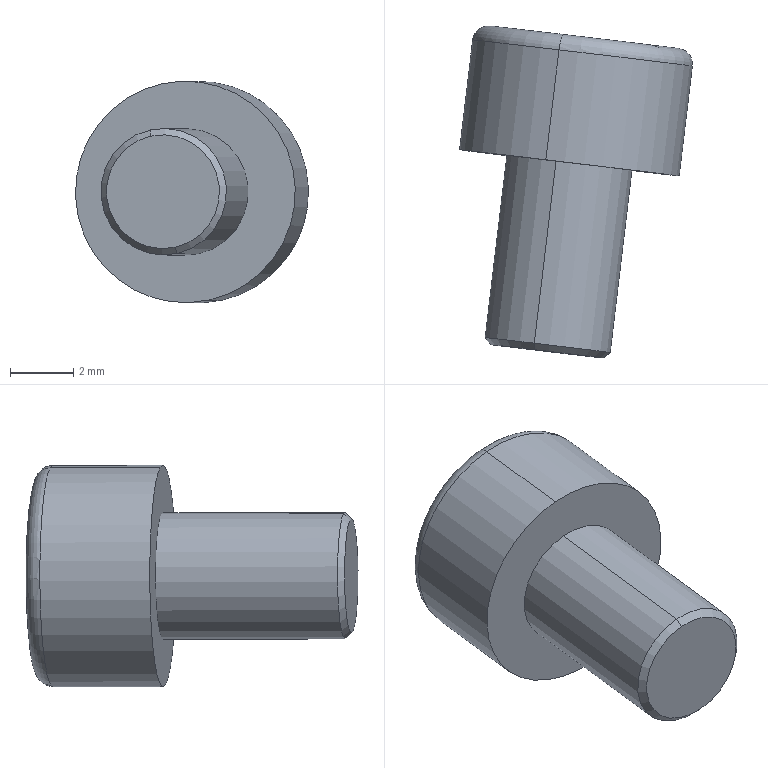Component | SolidWorks | hexagon socket head cap screws gb-5 | 1 solid | 25 faces | box 7.37 x 10.5 x 7 mm | volume 210 mm3 | plane 15 | cone 4 | cylinder 4 | torus 2 | commonest cylinder face diameters 4 x2 7 x2
STEP:
#1=CARTESIAN_POINT('',(0.04332,2.938,-0.1422));
#2=VERTEX_POINT('',#1);
#3=CARTESIAN_POINT('',(0.01319,2.942,-0.003732));
#4=VERTEX_POINT('',#3);
#5=CARTESIAN_POINT('',(0.02825,2.94,-0.07295));
#6=DIRECTION('',(-0.1183,-0.993,0.001159));
#7=DIRECTION('',(0.2126,-0.02647,-0.9768));
#8=AXIS2_PLACEMENT_3D('',#5,#6,#7);
#9=CIRCLE('',#8,0.07087);
#10=EDGE_CURVE('',#2,#4,#9,.T.);
#11=ORIENTED_EDGE('',*,*,#10,.F.);
#12=CARTESIAN_POINT('',(0.04593,2.946,-0.1499));
#13=VERTEX_POINT('',#12);
#14=CARTESIAN_POINT('',(0.04332,2.938,-0.1422));
#15=DIRECTION('',(0.234,0.6834,-0.6915));
#16=VECTOR('',#15,39.37);
#17=LINE('',#14,#16);
#18=EDGE_CURVE('',#2,#13,#17,.T.);
#19=ORIENTED_EDGE('',*,*,#18,.T.);
#20=CARTESIAN_POINT('',(0.01244,2.95,0.00395));
#21=VERTEX_POINT('',#20);
#22=CARTESIAN_POINT('',(0.02919,2.948,-0.07296));
#23=DIRECTION('',(0.1183,0.993,-0.001159));
#24=DIRECTION('',(0.2126,-0.02647,-0.9768));
#25=AXIS2_PLACEMENT_3D('',#22,#23,#24);
#26=CIRCLE('',#25,0.07874);
#27=EDGE_CURVE('',#21,#13,#26,.T.);
#28=ORIENTED_EDGE('',*,*,#27,.F.);
#29=CARTESIAN_POINT('',(0.01319,2.942,-0.003732));
#30=DIRECTION('',(-0.06668,0.7209,0.6899));
#31=VECTOR('',#30,39.37);
#32=LINE('',#29,#31);
#33=EDGE_CURVE('',#4,#21,#32,.T.);
#34=ORIENTED_EDGE('',*,*,#33,.F.);
#35=EDGE_LOOP('',(#11,#19,#28,#34));
#36=FACE_OUTER_BOUND('',#35,.T.);
#37=CARTESIAN_POINT('',(0.02825,2.94,-0.07295));
#38=DIRECTION('',(0.1183,0.993,-0.001159));
#39=DIRECTION('',(-0.2126,0.02647,0.9768));
#40=AXIS2_PLACEMENT_3D('',#37,#38,#39);
#41=CONICAL_SURFACE('',#40,0.07087,0.7854);
#42=ADVANCED_FACE('',(#36),#41,.T.);
#43=CARTESIAN_POINT('',(0.04972,3.334,0.04196));
#44=VERTEX_POINT('',#43);
#45=CARTESIAN_POINT('',(0.09995,3.328,-0.1888));
#46=VERTEX_POINT('',#45);
#47=CARTESIAN_POINT('',(0.07484,3.331,-0.07341));
#48=DIRECTION('',(0.1183,0.993,-0.001159));
#49=DIRECTION('',(0.2126,-0.02647,-0.9768));
#50=AXIS2_PLACEMENT_3D('',#47,#48,#49);
#51=CIRCLE('',#50,0.1181);
#52=EDGE_CURVE('',#44,#46,#51,.T.);
#53=ORIENTED_EDGE('',*,*,#52,.F.);
#54=CARTESIAN_POINT('',(0.04321,3.315,0.06121));
#55=VERTEX_POINT('',#54);
#56=CARTESIAN_POINT('',(0.0474,3.315,0.04198));
#57=DIRECTION('',(0.9699,-0.1153,0.2143));
#58=DIRECTION('',(0.2157,0.,-0.9765));
#59=AXIS2_PLACEMENT_3D('',#56,#57,#58);
#60=CIRCLE('',#59,0.01969);
#61=EDGE_CURVE('',#44,#55,#60,.T.);
#62=ORIENTED_EDGE('',*,*,#61,.T.);
#63=CARTESIAN_POINT('',(0.1018,3.308,-0.208));
#64=VERTEX_POINT('',#63);
#65=CARTESIAN_POINT('',(0.07251,3.312,-0.07339));
#66=DIRECTION('',(-0.1183,-0.993,0.001159));
#67=DIRECTION('',(0.2126,-0.02647,-0.9768));
#68=AXIS2_PLACEMENT_3D('',#65,#66,#67);
#69=CIRCLE('',#68,0.1378);
#70=EDGE_CURVE('',#64,#55,#69,.T.);
#71=ORIENTED_EDGE('',*,*,#70,.F.);
#72=CARTESIAN_POINT('',(0.09762,3.308,-0.1888));
#73=DIRECTION('',(-0.9699,0.1153,-0.2143));
#74=DIRECTION('',(-0.2157,0.,0.9765));
#75=AXIS2_PLACEMENT_3D('',#72,#73,#74);
#76=CIRCLE('',#75,0.01969);
#77=EDGE_CURVE('',#46,#64,#76,.T.);
#78=ORIENTED_EDGE('',*,*,#77,.F.);
#79=EDGE_LOOP('',(#53,#62,#71,#78));
#80=FACE_OUTER_BOUND('',#79,.T.);
#81=CARTESIAN_POINT('',(0.07251,3.312,-0.07339));
#82=DIRECTION('',(-0.1183,-0.993,0.001159));
#83=DIRECTION('',(0.2126,-0.02647,-0.9768));
#84=AXIS2_PLACEMENT_3D('',#81,#82,#83);
#85=TOROIDAL_SURFACE('',#84,0.1181,0.01969);
#86=ADVANCED_FACE('',(#80),#85,.T.);
#87=CARTESIAN_POINT('',(0.06149,3.219,-0.07328));
#88=VERTEX_POINT('',#87);
#89=CARTESIAN_POINT('',(0.05296,3.255,-0.01563));
#90=VERTEX_POINT('',#89);
#91=CARTESIAN_POINT('',(0.05296,3.255,-0.01563));
#92=DIRECTION('',(-0.125,0.5194,0.8453));
#93=VECTOR('',#92,39.37);
#94=LINE('',#91,#93);
#95=EDGE_CURVE('',#88,#90,#94,.T.);
#96=ORIENTED_EDGE('',*,*,#95,.F.);
#97=CARTESIAN_POINT('',(0.07808,3.251,-0.131));
#98=VERTEX_POINT('',#97);
#99=CARTESIAN_POINT('',(0.07808,3.251,-0.131));
#100=DIRECTION('',(0.2433,0.4736,-0.8465));
#101=VECTOR('',#100,39.37);
#102=LINE('',#99,#101);
#103=EDGE_CURVE('',#88,#98,#102,.T.);
#104=ORIENTED_EDGE('',*,*,#103,.T.);
#105=CARTESIAN_POINT('',(0.04775,3.255,-0.1296));
#106=VERTEX_POINT('',#105);
#107=CARTESIAN_POINT('',(0.06552,3.253,-0.07332));
#108=DIRECTION('',(-0.1183,-0.993,0.001159));
#109=DIRECTION('',(-0.2126,0.02647,0.9768));
#110=AXIS2_PLACEMENT_3D('',#107,#108,#109);
#111=CIRCLE('',#110,0.05906);
#112=EDGE_CURVE('',#106,#98,#111,.T.);
#113=ORIENTED_EDGE('',*,*,#112,.F.);
#114=CARTESIAN_POINT('',(0.00824,3.26,-0.08597));
#115=VERTEX_POINT('',#114);
#116=CARTESIAN_POINT('',(0.06552,3.253,-0.07332));
#117=DIRECTION('',(-0.1183,-0.993,0.001159));
#118=DIRECTION('',(-0.2126,0.02647,0.9768));
#119=AXIS2_PLACEMENT_3D('',#116,#117,#118);
#120=CIRCLE('',#119,0.05906);
#121=EDGE_CURVE('',#115,#106,#120,.T.);
#122=ORIENTED_EDGE('',*,*,#121,.F.);
#123=CARTESIAN_POINT('',(0.02601,3.258,-0.02969));
#124=VERTEX_POINT('',#123);
#125=CARTESIAN_POINT('',(0.06552,3.253,-0.07332));
#126=DIRECTION('',(-0.1183,-0.993,0.001159));
#127=DIRECTION('',(-0.2126,0.02647,0.9768));
#128=AXIS2_PLACEMENT_3D('',#125,#126,#127);
#129=CIRCLE('',#128,0.05906);
#130=EDGE_CURVE('',#124,#115,#129,.T.);
#131=ORIENTED_EDGE('',*,*,#130,.F.);
#132=CARTESIAN_POINT('',(0.06552,3.253,-0.07332));
#133=DIRECTION('',(-0.1183,-0.993,0.001159));
#134=DIRECTION('',(-0.2126,0.02647,0.9768));
#135=AXIS2_PLACEMENT_3D('',#132,#133,#134);
#136=CIRCLE('',#135,0.05906);
#137=EDGE_CURVE('',#90,#124,#136,.T.);
#138=ORIENTED_EDGE('',*,*,#137,.F.);
#139=EDGE_LOOP('',(#96,#104,#113,#122,#131,#138));
#140=FACE_OUTER_BOUND('',#139,.T.);
#141=CARTESIAN_POINT('',(0.06552,3.253,-0.07332));
#142=DIRECTION('',(0.1183,0.993,-0.001159));
#143=DIRECTION('',(-0.2126,0.02647,0.9768));
#144=AXIS2_PLACEMENT_3D('',#141,#142,#143);
#145=CONICAL_SURFACE('',#144,0.05906,1.047);
#146=ADVANCED_FACE('',(#140),#145,.F.);
#147=ORIENTED_EDGE('',*,*,#27,.T.);
#148=CARTESIAN_POINT('',(0.07294,3.173,-0.1501));
#149=VERTEX_POINT('',#148);
#150=CARTESIAN_POINT('',(0.045,2.938,-0.1499));
#151=DIRECTION('',(0.1183,0.993,-0.001159));
#152=VECTOR('',#151,39.37);
#153=LINE('',#150,#152);
#154=EDGE_CURVE('',#13,#149,#153,.T.);
#155=ORIENTED_EDGE('',*,*,#154,.T.);
#156=CARTESIAN_POINT('',(0.03946,3.177,0.003686));
#157=VERTEX_POINT('',#156);
#158=CARTESIAN_POINT('',(0.0562,3.175,-0.07323));
#159=DIRECTION('',(-0.1183,-0.993,0.001159));
#160=DIRECTION('',(0.2126,-0.02647,-0.9768));
#161=AXIS2_PLACEMENT_3D('',#158,#159,#160);
#162=CIRCLE('',#161,0.07874);
#163=EDGE_CURVE('',#149,#157,#162,.T.);
#164=ORIENTED_EDGE('',*,*,#163,.T.);
#165=CARTESIAN_POINT('',(0.01151,2.942,0.00396));
#166=DIRECTION('',(0.1183,0.993,-0.001159));
#167=VECTOR('',#166,39.37);
#168=LINE('',#165,#167);
#169=EDGE_CURVE('',#21,#157,#168,.T.);
#170=ORIENTED_EDGE('',*,*,#169,.F.);
#171=EDGE_LOOP('',(#147,#155,#164,#170));
#172=FACE_OUTER_BOUND('',#171,.T.);
#173=CARTESIAN_POINT('',(0.02825,2.94,-0.07295));
#174=DIRECTION('',(0.1183,0.993,-0.001159));
#175=DIRECTION('',(-0.2126,0.02647,0.9768));
#176=AXIS2_PLACEMENT_3D('',#173,#174,#175);
#177=CYLINDRICAL_SURFACE('',#176,0.07874);
#178=ADVANCED_FACE('',(#172),#177,.T.);
#179=CARTESIAN_POINT('',(0.0855,3.171,-0.2078));
#180=VERTEX_POINT('',#179);
#181=CARTESIAN_POINT('',(0.02691,3.178,0.06137));
#182=VERTEX_POINT('',#181);
#183=CARTESIAN_POINT('',(0.0562,3.175,-0.07323));
#184=DIRECTION('',(-0.1183,-0.993,0.001159));
#185=DIRECTION('',(0.2126,-0.02647,-0.9768));
#186=AXIS2_PLACEMENT_3D('',#183,#184,#185);
#187=CIRCLE('',#186,0.1378);
#188=EDGE_CURVE('',#180,#182,#187,.T.);
#189=ORIENTED_EDGE('',*,*,#188,.F.);
#190=CARTESIAN_POINT('',(0.0855,3.171,-0.2078));
#191=DIRECTION('',(0.1183,0.993,-0.001159));
#192=VECTOR('',#191,39.37);
#193=LINE('',#190,#192);
#194=EDGE_CURVE('',#180,#64,#193,.T.);
#195=ORIENTED_EDGE('',*,*,#194,.T.);
#196=ORIENTED_EDGE('',*,*,#70,.T.);
#197=CARTESIAN_POINT('',(0.02691,3.178,0.06137));
#198=DIRECTION('',(0.1183,0.993,-0.001159));
#199=VECTOR('',#198,39.37);
#200=LINE('',#197,#199);
#201=EDGE_CURVE('',#182,#55,#200,.T.);
#202=ORIENTED_EDGE('',*,*,#201,.F.);
#203=EDGE_LOOP('',(#189,#195,#196,#202));
#204=FACE_OUTER_BOUND('',#203,.T.);
#205=CARTESIAN_POINT('',(0.0562,3.175,-0.07323));
#206=DIRECTION('',(0.1183,0.993,-0.001159));
#207=DIRECTION('',(-0.2126,0.02647,0.9768));
#208=AXIS2_PLACEMENT_3D('',#205,#206,#207);
#209=CYLINDRICAL_SURFACE('',#208,0.1378);
#210=ADVANCED_FACE('',(#204),#209,.T.);
#211=CARTESIAN_POINT('',(0.0009904,3.261,-0.05267));
#212=VERTEX_POINT('',#211);
#213=CARTESIAN_POINT('',(0.05102,3.255,-0.00671));
#214=DIRECTION('',(-0.7337,0.08664,-0.6739));
#215=VECTOR('',#214,39.37);
#216=LINE('',#213,#215);
#217=EDGE_CURVE('',#124,#212,#216,.T.);
#218=ORIENTED_EDGE('',*,*,#217,.F.);
#219=ORIENTED_EDGE('',*,*,#130,.T.);
#220=CARTESIAN_POINT('',(0.0009904,3.261,-0.05267));
#221=DIRECTION('',(0.2126,-0.02647,-0.9768));
#222=VECTOR('',#221,39.37);
#223=LINE('',#220,#222);
#224=EDGE_CURVE('',#212,#115,#223,.T.);
#225=ORIENTED_EDGE('',*,*,#224,.F.);
#226=EDGE_LOOP('',(#218,#219,#225));
#227=FACE_OUTER_BOUND('',#226,.T.);
#228=CARTESIAN_POINT('',(-0.04904,3.267,-0.09862));
#229=DIRECTION('',(0.1183,0.993,-0.001159));
#230=DIRECTION('',(-0.2126,0.02647,0.9768));
#231=AXIS2_PLACEMENT_3D('',#228,#229,#230);
#232=PLANE('',#231);
#233=ADVANCED_FACE('',(#227),#232,.T.);
#234=CARTESIAN_POINT('',(0.01549,3.259,-0.1193));
#235=VERTEX_POINT('',#234);
#236=CARTESIAN_POINT('',(0.0009904,3.261,-0.05267));
#237=DIRECTION('',(0.2126,-0.02647,-0.9768));
#238=VECTOR('',#237,39.37);
#239=LINE('',#236,#238);
#240=EDGE_CURVE('',#115,#235,#239,.T.);
#241=ORIENTED_EDGE('',*,*,#240,.F.);
#242=ORIENTED_EDGE('',*,*,#121,.T.);
#243=CARTESIAN_POINT('',(0.01549,3.259,-0.1193));
#244=DIRECTION('',(0.9463,-0.1131,-0.3028));
#245=VECTOR('',#244,39.37);
#246=LINE('',#243,#245);
#247=EDGE_CURVE('',#235,#106,#246,.T.);
#248=ORIENTED_EDGE('',*,*,#247,.F.);
#249=EDGE_LOOP('',(#241,#242,#248));
#250=FACE_OUTER_BOUND('',#249,.T.);
#251=CARTESIAN_POINT('',(-0.04904,3.267,-0.09862));
#252=DIRECTION('',(0.1183,0.993,-0.001159));
#253=DIRECTION('',(-0.2126,0.02647,0.9768));
#254=AXIS2_PLACEMENT_3D('',#251,#252,#253);
#255=PLANE('',#254);
#256=ADVANCED_FACE('',(#250),#255,.T.);
#257=CARTESIAN_POINT('',(0.08002,3.251,-0.1399));
#258=VERTEX_POINT('',#257);
#259=CARTESIAN_POINT('',(0.01549,3.259,-0.1193));
#260=DIRECTION('',(0.9463,-0.1131,-0.3028));
#261=VECTOR('',#260,39.37);
#262=LINE('',#259,#261);
#263=EDGE_CURVE('',#106,#258,#262,.T.);
#264=ORIENTED_EDGE('',*,*,#263,.F.);
#265=ORIENTED_EDGE('',*,*,#112,.T.);
#266=CARTESIAN_POINT('',(0.105,3.248,-0.1169));
#267=VERTEX_POINT('',#266);
#268=CARTESIAN_POINT('',(0.06552,3.253,-0.07332));
#269=DIRECTION('',(-0.1183,-0.993,0.001159));
#270=DIRECTION('',(-0.2126,0.02647,0.9768));
#271=AXIS2_PLACEMENT_3D('',#268,#269,#270);
#272=CIRCLE('',#271,0.05906);
#273=EDGE_CURVE('',#98,#267,#272,.T.);
#274=ORIENTED_EDGE('',*,*,#273,.T.);
#275=CARTESIAN_POINT('',(0.08002,3.251,-0.1399));
#276=DIRECTION('',(0.7337,-0.08664,0.6739));
#277=VECTOR('',#276,39.37);
#278=LINE('',#275,#277);
#279=EDGE_CURVE('',#258,#267,#278,.T.);
#280=ORIENTED_EDGE('',*,*,#279,.F.);
#281=EDGE_LOOP('',(#264,#265,#274,#280));
#282=FACE_OUTER_BOUND('',#281,.T.);
#283=CARTESIAN_POINT('',(-0.04904,3.267,-0.09862));
#284=DIRECTION('',(0.1183,0.993,-0.001159));
#285=DIRECTION('',(-0.2126,0.02647,0.9768));
#286=AXIS2_PLACEMENT_3D('',#283,#284,#285);
#287=PLANE('',#286);
#288=ADVANCED_FACE('',(#282),#287,.T.);
#289=CARTESIAN_POINT('',(0.13,3.245,-0.09397));
#290=VERTEX_POINT('',#289);
#291=CARTESIAN_POINT('',(0.08002,3.251,-0.1399));
#292=DIRECTION('',(0.7337,-0.08664,0.6739));
#293=VECTOR('',#292,39.37);
#294=LINE('',#291,#293);
#295=EDGE_CURVE('',#267,#290,#294,.T.);
#296=ORIENTED_EDGE('',*,*,#295,.F.);
#297=CARTESIAN_POINT('',(0.1228,3.246,-0.06066));
#298=VERTEX_POINT('',#297);
#299=CARTESIAN_POINT('',(0.06552,3.253,-0.07332));
#300=DIRECTION('',(-0.1183,-0.993,0.001159));
#301=DIRECTION('',(0.2126,-0.02647,-0.9768));
#302=AXIS2_PLACEMENT_3D('',#299,#300,#301);
#303=CIRCLE('',#302,0.05906);
#304=EDGE_CURVE('',#267,#298,#303,.T.);
#305=ORIENTED_EDGE('',*,*,#304,.T.);
#306=CARTESIAN_POINT('',(0.13,3.245,-0.09397));
#307=DIRECTION('',(-0.2126,0.02647,0.9768));
#308=VECTOR('',#307,39.37);
#309=LINE('',#306,#308);
#310=EDGE_CURVE('',#290,#298,#309,.T.);
#311=ORIENTED_EDGE('',*,*,#310,.F.);
#312=EDGE_LOOP('',(#296,#305,#311));
#313=FACE_OUTER_BOUND('',#312,.T.);
#314=CARTESIAN_POINT('',(-0.04904,3.267,-0.09862));
#315=DIRECTION('',(0.1183,0.993,-0.001159));
#316=DIRECTION('',(-0.2126,0.02647,0.9768));
#317=AXIS2_PLACEMENT_3D('',#314,#315,#316);
#318=PLANE('',#317);
#319=ADVANCED_FACE('',(#313),#318,.T.);
#320=CARTESIAN_POINT('',(0.1156,3.247,-0.02736));
#321=VERTEX_POINT('',#320);
#322=CARTESIAN_POINT('',(0.13,3.245,-0.09397));
#323=DIRECTION('',(-0.2126,0.02647,0.9768));
#324=VECTOR('',#323,39.37);
#325=LINE('',#322,#324);
#326=EDGE_CURVE('',#298,#321,#325,.T.);
#327=ORIENTED_EDGE('',*,*,#326,.F.);
#328=CARTESIAN_POINT('',(0.08329,3.251,-0.01704));
#329=VERTEX_POINT('',#328);
#330=CARTESIAN_POINT('',(0.06552,3.253,-0.07332));
#331=DIRECTION('',(-0.1183,-0.993,0.001159));
#332=DIRECTION('',(-0.2126,0.02647,0.9768));
#333=AXIS2_PLACEMENT_3D('',#330,#331,#332);
#334=CIRCLE('',#333,0.05906);
#335=EDGE_CURVE('',#298,#329,#334,.T.);
#336=ORIENTED_EDGE('',*,*,#335,.T.);
#337=CARTESIAN_POINT('',(0.1156,3.247,-0.02736));
#338=DIRECTION('',(-0.9463,0.1131,0.3028));
#339=VECTOR('',#338,39.37);
#340=LINE('',#337,#339);
#341=EDGE_CURVE('',#321,#329,#340,.T.);
#342=ORIENTED_EDGE('',*,*,#341,.F.);
#343=EDGE_LOOP('',(#327,#336,#342));
#344=FACE_OUTER_BOUND('',#343,.T.);
#345=CARTESIAN_POINT('',(-0.04904,3.267,-0.09862));
#346=DIRECTION('',(0.1183,0.993,-0.001159));
#347=DIRECTION('',(-0.2126,0.02647,0.9768));
#348=AXIS2_PLACEMENT_3D('',#345,#346,#347);
#349=PLANE('',#348);
#350=ADVANCED_FACE('',(#344),#349,.T.);
#351=CARTESIAN_POINT('',(0.05102,3.255,-0.00671));
#352=VERTEX_POINT('',#351);
#353=CARTESIAN_POINT('',(0.1156,3.247,-0.02736));
#354=DIRECTION('',(-0.9463,0.1131,0.3028));
#355=VECTOR('',#354,39.37);
#356=LINE('',#353,#355);
#357=EDGE_CURVE('',#329,#352,#356,.T.);
#358=ORIENTED_EDGE('',*,*,#357,.F.);
#359=CARTESIAN_POINT('',(0.06552,3.253,-0.07332));
#360=DIRECTION('',(-0.1183,-0.993,0.001159));
#361=DIRECTION('',(-0.2126,0.02647,0.9768));
#362=AXIS2_PLACEMENT_3D('',#359,#360,#361);
#363=CIRCLE('',#362,0.05906);
#364=EDGE_CURVE('',#329,#90,#363,.T.);
#365=ORIENTED_EDGE('',*,*,#364,.T.);
#366=ORIENTED_EDGE('',*,*,#137,.T.);
#367=CARTESIAN_POINT('',(0.05102,3.255,-0.00671));
#368=DIRECTION('',(-0.7337,0.08664,-0.6739));
#369=VECTOR('',#368,39.37);
#370=LINE('',#367,#369);
#371=EDGE_CURVE('',#352,#124,#370,.T.);
#372=ORIENTED_EDGE('',*,*,#371,.F.);
#373=EDGE_LOOP('',(#358,#365,#366,#372));
#374=FACE_OUTER_BOUND('',#373,.T.);
#375=CARTESIAN_POINT('',(-0.04904,3.267,-0.09862));
#376=DIRECTION('',(0.1183,0.993,-0.001159));
#377=DIRECTION('',(-0.2126,0.02647,0.9768));
#378=AXIS2_PLACEMENT_3D('',#375,#376,#377);
#379=PLANE('',#378);
#380=ADVANCED_FACE('',(#374),#379,.T.);
#381=CARTESIAN_POINT('',(0.07484,3.331,-0.07341));
#382=DIRECTION('',(0.1183,0.993,-0.001159));
#383=DIRECTION('',(0.2126,-0.02647,-0.9768));
#384=AXIS2_PLACEMENT_3D('',#381,#382,#383);
#385=CIRCLE('',#384,0.1181);
#386=EDGE_CURVE('',#46,#44,#385,.T.);
#387=ORIENTED_EDGE('',*,*,#386,.T.);
#388=ORIENTED_EDGE('',*,*,#52,.T.);
#389=EDGE_LOOP('',(#387,#388));
#390=FACE_OUTER_BOUND('',#389,.T.);
#391=CARTESIAN_POINT('',(0.02481,3.337,-0.1194));
#392=VERTEX_POINT('',#391);
#393=CARTESIAN_POINT('',(0.08933,3.329,-0.14));
#394=VERTEX_POINT('',#393);
#395=CARTESIAN_POINT('',(0.02481,3.337,-0.1194));
#396=DIRECTION('',(0.9463,-0.1131,-0.3028));
#397=VECTOR('',#396,39.37);
#398=LINE('',#395,#397);
#399=EDGE_CURVE('',#392,#394,#398,.T.);
#400=ORIENTED_EDGE('',*,*,#399,.T.);
#401=CARTESIAN_POINT('',(0.1394,3.323,-0.09406));
#402=VERTEX_POINT('',#401);
#403=CARTESIAN_POINT('',(0.08933,3.329,-0.14));
#404=DIRECTION('',(0.7337,-0.08664,0.6739));
#405=VECTOR('',#404,39.37);
#406=LINE('',#403,#405);
#407=EDGE_CURVE('',#394,#402,#406,.T.);
#408=ORIENTED_EDGE('',*,*,#407,.T.);
#409=CARTESIAN_POINT('',(0.1249,3.325,-0.02745));
#410=VERTEX_POINT('',#409);
#411=CARTESIAN_POINT('',(0.1394,3.323,-0.09406));
#412=DIRECTION('',(-0.2126,0.02647,0.9768));
#413=VECTOR('',#412,39.37);
#414=LINE('',#411,#413);
#415=EDGE_CURVE('',#402,#410,#414,.T.);
#416=ORIENTED_EDGE('',*,*,#415,.T.);
#417=CARTESIAN_POINT('',(0.06034,3.333,-0.006801));
#418=VERTEX_POINT('',#417);
#419=CARTESIAN_POINT('',(0.1249,3.325,-0.02745));
#420=DIRECTION('',(-0.9463,0.1131,0.3028));
#421=VECTOR('',#420,39.37);
#422=LINE('',#419,#421);
#423=EDGE_CURVE('',#410,#418,#422,.T.);
#424=ORIENTED_EDGE('',*,*,#423,.T.);
#425=CARTESIAN_POINT('',(0.01031,3.339,-0.05276));
#426=VERTEX_POINT('',#425);
#427=CARTESIAN_POINT('',(0.06034,3.333,-0.006801));
#428=DIRECTION('',(-0.7337,0.08664,-0.6739));
#429=VECTOR('',#428,39.37);
#430=LINE('',#427,#429);
#431=EDGE_CURVE('',#418,#426,#430,.T.);
#432=ORIENTED_EDGE('',*,*,#431,.T.);
#433=CARTESIAN_POINT('',(0.01031,3.339,-0.05276));
#434=DIRECTION('',(0.2126,-0.02647,-0.9768));
#435=VECTOR('',#434,39.37);
#436=LINE('',#433,#435);
#437=EDGE_CURVE('',#426,#392,#436,.T.);
#438=ORIENTED_EDGE('',*,*,#437,.T.);
#439=EDGE_LOOP('',(#400,#408,#416,#424,#432,#438));
#440=FACE_BOUND('',#439,.T.);
#441=CARTESIAN_POINT('',(0.07484,3.331,-0.07341));
#442=DIRECTION('',(-0.1183,-0.993,0.001159));
#443=DIRECTION('',(0.2126,-0.02647,-0.9768));
#444=AXIS2_PLACEMENT_3D('',#441,#442,#443);
#445=PLANE('',#444);
#446=ADVANCED_FACE('',(#390,#440),#445,.F.);
#447=CARTESIAN_POINT('',(0.0562,3.175,-0.07323));
#448=DIRECTION('',(-0.1183,-0.993,0.001159));
#449=DIRECTION('',(0.2126,-0.02647,-0.9768));
#450=AXIS2_PLACEMENT_3D('',#447,#448,#449);
#451=CIRCLE('',#450,0.1378);
#452=EDGE_CURVE('',#182,#180,#451,.T.);
#453=ORIENTED_EDGE('',*,*,#452,.T.);
#454=ORIENTED_EDGE('',*,*,#188,.T.);
#455=EDGE_LOOP('',(#453,#454));
#456=FACE_OUTER_BOUND('',#455,.T.);
#457=CARTESIAN_POINT('',(0.0562,3.175,-0.07323));
#458=DIRECTION('',(-0.1183,-0.993,0.001159));
#459=DIRECTION('',(0.2126,-0.02647,-0.9768));
#460=AXIS2_PLACEMENT_3D('',#457,#458,#459);
#461=CIRCLE('',#460,0.07874);
#462=EDGE_CURVE('',#157,#149,#461,.T.);
#463=ORIENTED_EDGE('',*,*,#462,.F.);
#464=ORIENTED_EDGE('',*,*,#163,.F.);
#465=EDGE_LOOP('',(#463,#464));
#466=FACE_BOUND('',#465,.T.);
#467=CARTESIAN_POINT('',(0.0562,3.175,-0.07323));
#468=DIRECTION('',(-0.1183,-0.993,0.001159));
#469=DIRECTION('',(0.2126,-0.02647,-0.9768));
#470=AXIS2_PLACEMENT_3D('',#467,#468,#469);
#471=PLANE('',#470);
#472=ADVANCED_FACE('',(#456,#466),#471,.T.);
#473=ORIENTED_EDGE('',*,*,#194,.F.);
#474=ORIENTED_EDGE('',*,*,#452,.F.);
#475=ORIENTED_EDGE('',*,*,#201,.T.);
#476=CARTESIAN_POINT('',(0.07251,3.312,-0.07339));
#477=DIRECTION('',(-0.1183,-0.993,0.001159));
#478=DIRECTION('',(0.2126,-0.02647,-0.9768));
#479=AXIS2_PLACEMENT_3D('',#476,#477,#478);
#480=CIRCLE('',#479,0.1378);
#481=EDGE_CURVE('',#55,#64,#480,.T.);
#482=ORIENTED_EDGE('',*,*,#481,.T.);
#483=EDGE_LOOP('',(#473,#474,#475,#482));
#484=FACE_OUTER_BOUND('',#483,.T.);
#485=CARTESIAN_POINT('',(0.0562,3.175,-0.07323));
#486=DIRECTION('',(0.1183,0.993,-0.001159));
#487=DIRECTION('',(-0.2126,0.02647,0.9768));
#488=AXIS2_PLACEMENT_3D('',#485,#486,#487);
#489=CYLINDRICAL_SURFACE('',#488,0.1378);
#490=ADVANCED_FACE('',(#484),#489,.T.);
#491=ORIENTED_EDGE('',*,*,#154,.F.);
#492=CARTESIAN_POINT('',(0.02919,2.948,-0.07296));
#493=DIRECTION('',(0.1183,0.993,-0.001159));
#494=DIRECTION('',(0.2126,-0.02647,-0.9768));
#495=AXIS2_PLACEMENT_3D('',#492,#493,#494);
#496=CIRCLE('',#495,0.07874);
#497=EDGE_CURVE('',#13,#21,#496,.T.);
#498=ORIENTED_EDGE('',*,*,#497,.T.);
#499=ORIENTED_EDGE('',*,*,#169,.T.);
#500=ORIENTED_EDGE('',*,*,#462,.T.);
#501=EDGE_LOOP('',(#491,#498,#499,#500));
#502=FACE_OUTER_BOUND('',#501,.T.);
#503=CARTESIAN_POINT('',(0.02825,2.94,-0.07295));
#504=DIRECTION('',(0.1183,0.993,-0.001159));
#505=DIRECTION('',(-0.2126,0.02647,0.9768));
#506=AXIS2_PLACEMENT_3D('',#503,#504,#505);
#507=CYLINDRICAL_SURFACE('',#506,0.07874);
#508=ADVANCED_FACE('',(#502),#507,.T.);
#509=CARTESIAN_POINT('',(0.02825,2.94,-0.07295));
#510=DIRECTION('',(-0.1183,-0.993,0.001159));
#511=DIRECTION('',(0.2126,-0.02647,-0.9768));
#512=AXIS2_PLACEMENT_3D('',#509,#510,#511);
#513=CIRCLE('',#512,0.07087);
#514=EDGE_CURVE('',#4,#2,#513,.T.);
#515=ORIENTED_EDGE('',*,*,#514,.T.);
#516=ORIENTED_EDGE('',*,*,#10,.T.);
#517=EDGE_LOOP('',(#515,#516));
#518=FACE_OUTER_BOUND('',#517,.T.);
#519=CARTESIAN_POINT('',(0.02825,2.94,-0.07295));
#520=DIRECTION('',(-0.1183,-0.993,0.001159));
#521=DIRECTION('',(0.2126,-0.02647,-0.9768));
#522=AXIS2_PLACEMENT_3D('',#519,#520,#521);
#523=PLANE('',#522);
#524=ADVANCED_FACE('',(#518),#523,.T.);
#525=ORIENTED_EDGE('',*,*,#399,.F.);
#526=CARTESIAN_POINT('',(0.01549,3.259,-0.1193));
#527=DIRECTION('',(0.1183,0.993,-0.001159));
#528=VECTOR('',#527,39.37);
#529=LINE('',#526,#528);
#530=EDGE_CURVE('',#235,#392,#529,.T.);
#531=ORIENTED_EDGE('',*,*,#530,.F.);
#532=ORIENTED_EDGE('',*,*,#247,.T.);
#533=ORIENTED_EDGE('',*,*,#263,.T.);
#534=CARTESIAN_POINT('',(0.08002,3.251,-0.1399));
#535=DIRECTION('',(0.1183,0.993,-0.001159));
#536=VECTOR('',#535,39.37);
#537=LINE('',#534,#536);
#538=EDGE_CURVE('',#258,#394,#537,.T.);
#539=ORIENTED_EDGE('',*,*,#538,.T.);
#540=EDGE_LOOP('',(#525,#531,#532,#533,#539));
#541=FACE_OUTER_BOUND('',#540,.T.);
#542=CARTESIAN_POINT('',(0.01549,3.259,-0.1193));
#543=DIRECTION('',(0.3008,-0.03474,0.953));
#544=DIRECTION('',(-0.9463,0.1131,0.3028));
#545=AXIS2_PLACEMENT_3D('',#542,#543,#544);
#546=PLANE('',#545);
#547=ADVANCED_FACE('',(#541),#546,.T.);
#548=ORIENTED_EDGE('',*,*,#407,.F.);
#549=ORIENTED_EDGE('',*,*,#538,.F.);
#550=ORIENTED_EDGE('',*,*,#279,.T.);
#551=ORIENTED_EDGE('',*,*,#295,.T.);
#552=CARTESIAN_POINT('',(0.13,3.245,-0.09397));
#553=DIRECTION('',(0.1183,0.993,-0.001159));
#554=VECTOR('',#553,39.37);
#555=LINE('',#552,#554);
#556=EDGE_CURVE('',#290,#402,#555,.T.);
#557=ORIENTED_EDGE('',*,*,#556,.T.);
#558=EDGE_LOOP('',(#548,#549,#550,#551,#557));
#559=FACE_OUTER_BOUND('',#558,.T.);
#560=CARTESIAN_POINT('',(0.08002,3.251,-0.1399));
#561=DIRECTION('',(-0.6691,0.08059,0.7388));
#562=DIRECTION('',(-0.7337,0.08664,-0.6739));
#563=AXIS2_PLACEMENT_3D('',#560,#561,#562);
#564=PLANE('',#563);
#565=ADVANCED_FACE('',(#559),#564,.T.);
#566=ORIENTED_EDGE('',*,*,#415,.F.);
#567=ORIENTED_EDGE('',*,*,#556,.F.);
#568=ORIENTED_EDGE('',*,*,#310,.T.);
#569=ORIENTED_EDGE('',*,*,#326,.T.);
#570=CARTESIAN_POINT('',(0.1156,3.247,-0.02736));
#571=DIRECTION('',(0.1183,0.993,-0.001159));
#572=VECTOR('',#571,39.37);
#573=LINE('',#570,#572);
#574=EDGE_CURVE('',#321,#410,#573,.T.);
#575=ORIENTED_EDGE('',*,*,#574,.T.);
#576=EDGE_LOOP('',(#566,#567,#568,#569,#575));
#577=FACE_OUTER_BOUND('',#576,.T.);
#578=CARTESIAN_POINT('',(0.13,3.245,-0.09397));
#579=DIRECTION('',(-0.9699,0.1153,-0.2143));
#580=DIRECTION('',(0.2126,-0.02647,-0.9768));
#581=AXIS2_PLACEMENT_3D('',#578,#579,#580);
#582=PLANE('',#581);
#583=ADVANCED_FACE('',(#577),#582,.T.);
#584=ORIENTED_EDGE('',*,*,#423,.F.);
#585=ORIENTED_EDGE('',*,*,#574,.F.);
#586=ORIENTED_EDGE('',*,*,#341,.T.);
#587=ORIENTED_EDGE('',*,*,#357,.T.);
#588=CARTESIAN_POINT('',(0.05102,3.255,-0.00671));
#589=DIRECTION('',(0.1183,0.993,-0.001159));
#590=VECTOR('',#589,39.37);
#591=LINE('',#588,#590);
#592=EDGE_CURVE('',#352,#418,#591,.T.);
#593=ORIENTED_EDGE('',*,*,#592,.T.);
#594=EDGE_LOOP('',(#584,#585,#586,#587,#593));
#595=FACE_OUTER_BOUND('',#594,.T.);
#596=CARTESIAN_POINT('',(0.1156,3.247,-0.02736));
#597=DIRECTION('',(-0.3008,0.03474,-0.953));
#598=DIRECTION('',(0.9463,-0.1131,-0.3028));
#599=AXIS2_PLACEMENT_3D('',#596,#597,#598);
#600=PLANE('',#599);
#601=ADVANCED_FACE('',(#595),#600,.T.);
#602=ORIENTED_EDGE('',*,*,#431,.F.);
#603=ORIENTED_EDGE('',*,*,#592,.F.);
#604=ORIENTED_EDGE('',*,*,#371,.T.);
#605=ORIENTED_EDGE('',*,*,#217,.T.);
#606=CARTESIAN_POINT('',(0.0009904,3.261,-0.05267));
#607=DIRECTION('',(0.1183,0.993,-0.001159));
#608=VECTOR('',#607,39.37);
#609=LINE('',#606,#608);
#610=EDGE_CURVE('',#212,#426,#609,.T.);
#611=ORIENTED_EDGE('',*,*,#610,.T.);
#612=EDGE_LOOP('',(#602,#603,#604,#605,#611));
#613=FACE_OUTER_BOUND('',#612,.T.);
#614=CARTESIAN_POINT('',(0.05102,3.255,-0.00671));
#615=DIRECTION('',(0.6691,-0.08059,-0.7388));
#616=DIRECTION('',(0.7337,-0.08664,0.6739));
#617=AXIS2_PLACEMENT_3D('',#614,#615,#616);
#618=PLANE('',#617);
#619=ADVANCED_FACE('',(#613),#618,.T.);
#620=ORIENTED_EDGE('',*,*,#437,.F.);
#621=ORIENTED_EDGE('',*,*,#610,.F.);
#622=ORIENTED_EDGE('',*,*,#224,.T.);
#623=ORIENTED_EDGE('',*,*,#240,.T.);
#624=ORIENTED_EDGE('',*,*,#530,.T.);
#625=EDGE_LOOP('',(#620,#621,#622,#623,#624));
#626=FACE_OUTER_BOUND('',#625,.T.);
#627=CARTESIAN_POINT('',(0.0009904,3.261,-0.05267));
#628=DIRECTION('',(0.9699,-0.1153,0.2143));
#629=DIRECTION('',(-0.2126,0.02647,0.9768));
#630=AXIS2_PLACEMENT_3D('',#627,#628,#629);
#631=PLANE('',#630);
#632=ADVANCED_FACE('',(#626),#631,.T.);
#633=ORIENTED_EDGE('',*,*,#103,.F.);
#634=ORIENTED_EDGE('',*,*,#95,.T.);
#635=ORIENTED_EDGE('',*,*,#364,.F.);
#636=ORIENTED_EDGE('',*,*,#335,.F.);
#637=ORIENTED_EDGE('',*,*,#304,.F.);
#638=ORIENTED_EDGE('',*,*,#273,.F.);
#639=EDGE_LOOP('',(#633,#634,#635,#636,#637,#638));
#640=FACE_OUTER_BOUND('',#639,.T.);
#641=CARTESIAN_POINT('',(0.06552,3.253,-0.07332));
#642=DIRECTION('',(0.1183,0.993,-0.001159));
#643=DIRECTION('',(-0.2126,0.02647,0.9768));
#644=AXIS2_PLACEMENT_3D('',#641,#642,#643);
#645=CONICAL_SURFACE('',#644,0.05906,1.047);
#646=ADVANCED_FACE('',(#640),#645,.F.);
#647=ORIENTED_EDGE('',*,*,#61,.F.);
#648=ORIENTED_EDGE('',*,*,#386,.F.);
#649=ORIENTED_EDGE('',*,*,#77,.T.);
#650=ORIENTED_EDGE('',*,*,#481,.F.);
#651=EDGE_LOOP('',(#647,#648,#649,#650));
#652=FACE_OUTER_BOUND('',#651,.T.);
#653=CARTESIAN_POINT('',(0.07251,3.312,-0.07339));
#654=DIRECTION('',(-0.1183,-0.993,0.001159));
#655=DIRECTION('',(0.2126,-0.02647,-0.9768));
#656=AXIS2_PLACEMENT_3D('',#653,#654,#655);
#657=TOROIDAL_SURFACE('',#656,0.1181,0.01969);
#658=ADVANCED_FACE('',(#652),#657,.T.);
#659=ORIENTED_EDGE('',*,*,#18,.F.);
#660=ORIENTED_EDGE('',*,*,#514,.F.);
#661=ORIENTED_EDGE('',*,*,#33,.T.);
#662=ORIENTED_EDGE('',*,*,#497,.F.);
#663=EDGE_LOOP('',(#659,#660,#661,#662));
#664=FACE_OUTER_BOUND('',#663,.T.);
#665=CARTESIAN_POINT('',(0.02825,2.94,-0.07295));
#666=DIRECTION('',(0.1183,0.993,-0.001159));
#667=DIRECTION('',(-0.2126,0.02647,0.9768));
#668=AXIS2_PLACEMENT_3D('',#665,#666,#667);
#669=CONICAL_SURFACE('',#668,0.07087,0.7854);
#670=ADVANCED_FACE('',(#664),#669,.T.);
#671=CLOSED_SHELL('',(#42,#86,#146,#178,#210,#233,#256,#288,#319,#350,#380,#446,#472,#490,#508,#524,#547,#565,#583,#601,#619,#632,#646,#658,#670));
#672=MANIFOLD_SOLID_BREP('',#671);
#673=CARTESIAN_POINT('',(0.,0.,0.));
#674=DIRECTION('',(0.,0.,1.));
#675=DIRECTION('',(1.,0.,0.));
#676=AXIS2_PLACEMENT_3D('',#673,#674,#675);
#677=(LENGTH_UNIT()NAMED_UNIT(*)SI_UNIT($,.METRE.));
#678=LENGTH_MEASURE_WITH_UNIT(LENGTH_MEASURE(0.0254),#677);
#679=DIMENSIONAL_EXPONENTS(1.,0.,0.,0.,0.,0.,0.);
#680=(CONVERSION_BASED_UNIT('',#678)LENGTH_UNIT()NAMED_UNIT(#679));
#681=UNCERTAINTY_MEASURE_WITH_UNIT(LENGTH_MEASURE(0.00001),#680,'','');
#682=(NAMED_UNIT(*)PLANE_ANGLE_UNIT()SI_UNIT($,.RADIAN.));
#683=(NAMED_UNIT(*)SI_UNIT($,.STERADIAN.)SOLID_ANGLE_UNIT());
#684=(GEOMETRIC_REPRESENTATION_CONTEXT(3)GLOBAL_UNCERTAINTY_ASSIGNED_CONTEXT((#681))GLOBAL_UNIT_ASSIGNED_CONTEXT((#680,#682,#683))REPRESENTATION_CONTEXT('',''));
#685=ADVANCED_BREP_SHAPE_REPRESENTATION('',(#672,#676),#684);
#686=COLOUR_RGB('',0.7922,0.8196,0.9333);
#687=FILL_AREA_STYLE_COLOUR('',#686);
#688=FILL_AREA_STYLE('',(#687));
#689=SURFACE_STYLE_FILL_AREA(#688);
#690=SURFACE_SIDE_STYLE('',(#689));
#691=SURFACE_STYLE_USAGE(.BOTH.,#690);
#692=PRESENTATION_STYLE_ASSIGNMENT((#691));
#693=STYLED_ITEM('',(#692),#672);
#694=(LENGTH_UNIT()NAMED_UNIT(*)SI_UNIT($,.METRE.));
#695=LENGTH_MEASURE_WITH_UNIT(LENGTH_MEASURE(0.0254),#694);
#696=DIMENSIONAL_EXPONENTS(1.,0.,0.,0.,0.,0.,0.);
#697=(CONVERSION_BASED_UNIT('',#695)LENGTH_UNIT()NAMED_UNIT(#696));
#698=UNCERTAINTY_MEASURE_WITH_UNIT(LENGTH_MEASURE(0.00001),#697,'','');
#699=(NAMED_UNIT(*)PLANE_ANGLE_UNIT()SI_UNIT($,.RADIAN.));
#700=(NAMED_UNIT(*)SI_UNIT($,.STERADIAN.)SOLID_ANGLE_UNIT());
#701=(GEOMETRIC_REPRESENTATION_CONTEXT(3)GLOBAL_UNCERTAINTY_ASSIGNED_CONTEXT((#698))GLOBAL_UNIT_ASSIGNED_CONTEXT((#697,#699,#700))REPRESENTATION_CONTEXT('',''));
#702=MECHANICAL_DESIGN_GEOMETRIC_PRESENTATION_REPRESENTATION('',(#693),#701);
#703=PRESENTATION_LAYER_ASSIGNMENT('','',(#693));